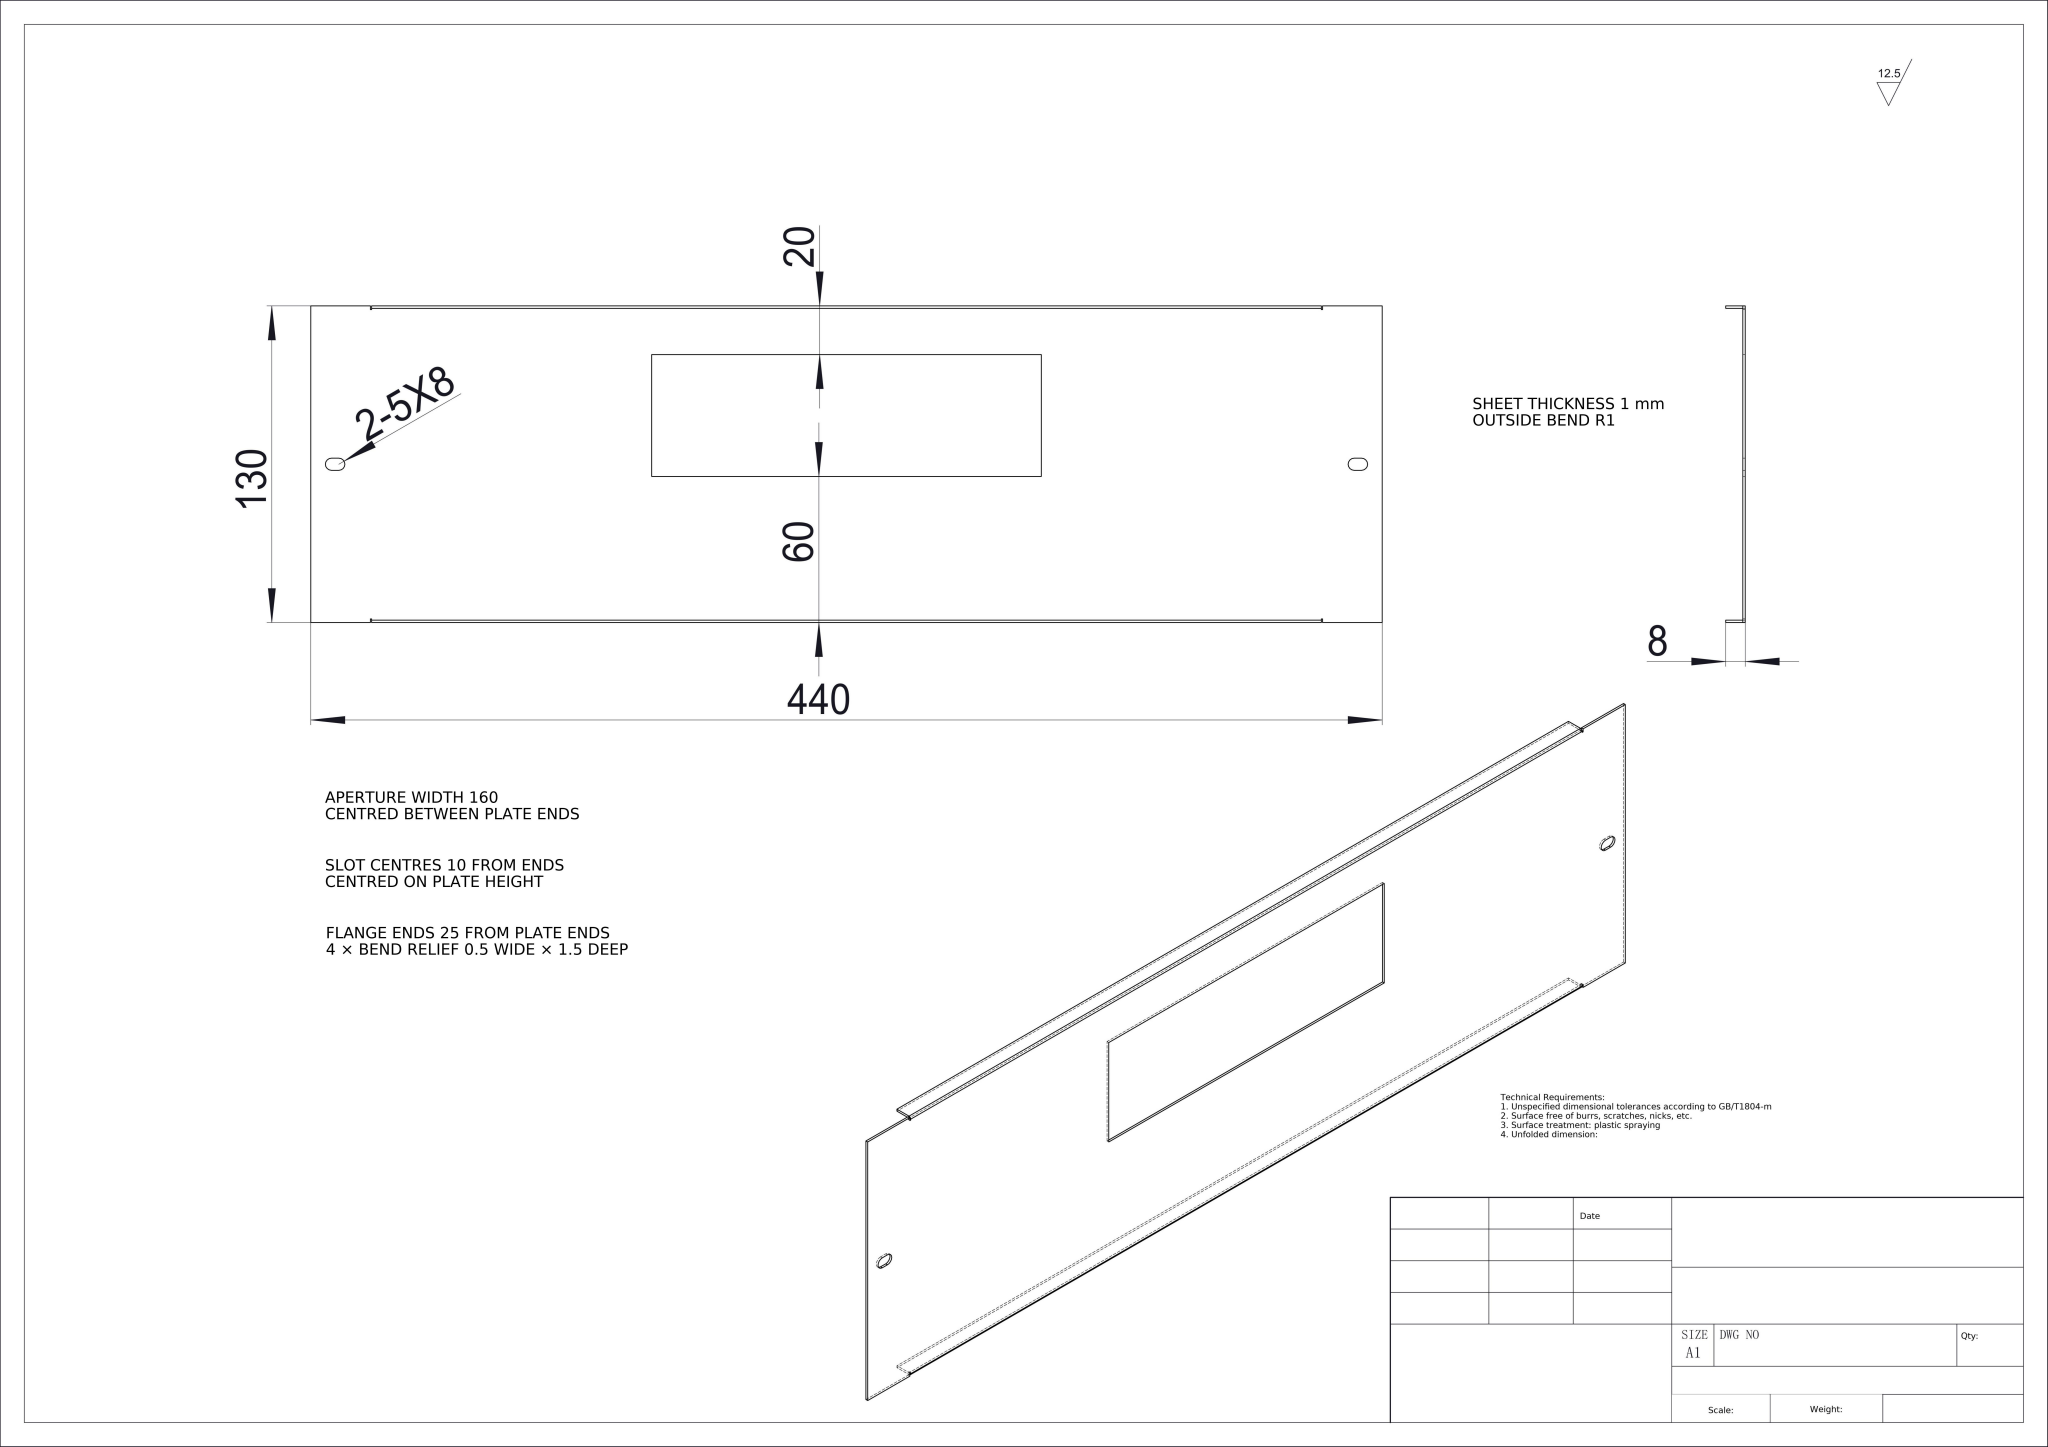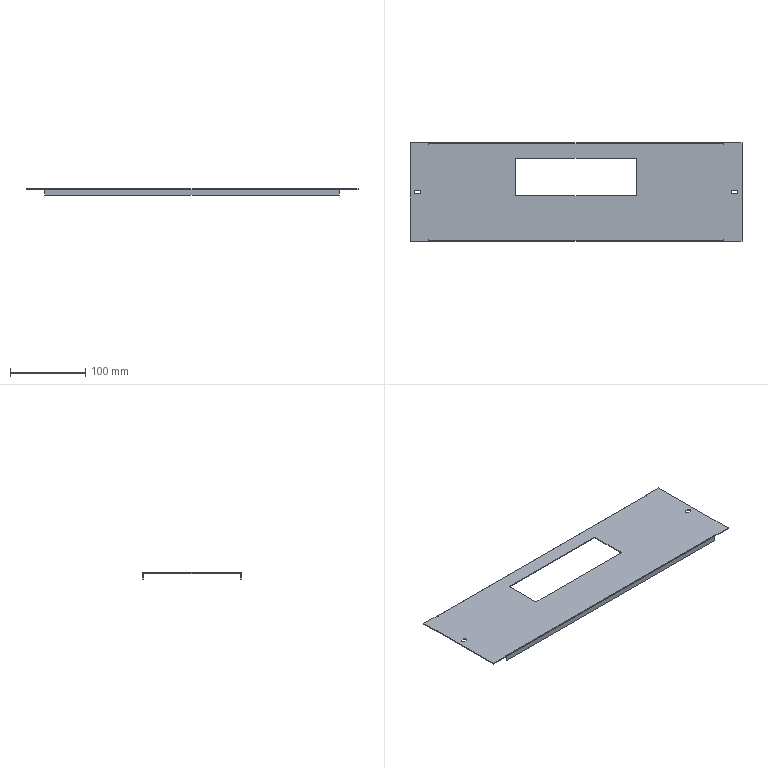Part | NX | mm | Rectangular Access Panel With Offset Rectangular Aperture 440mm | 1 solid | 50 faces | box 440 x 130 x 8 mm | volume 54420 mm3 | plane 42 | cylinder 8 | commonest cylinder face diameters 5 x6 2 x2